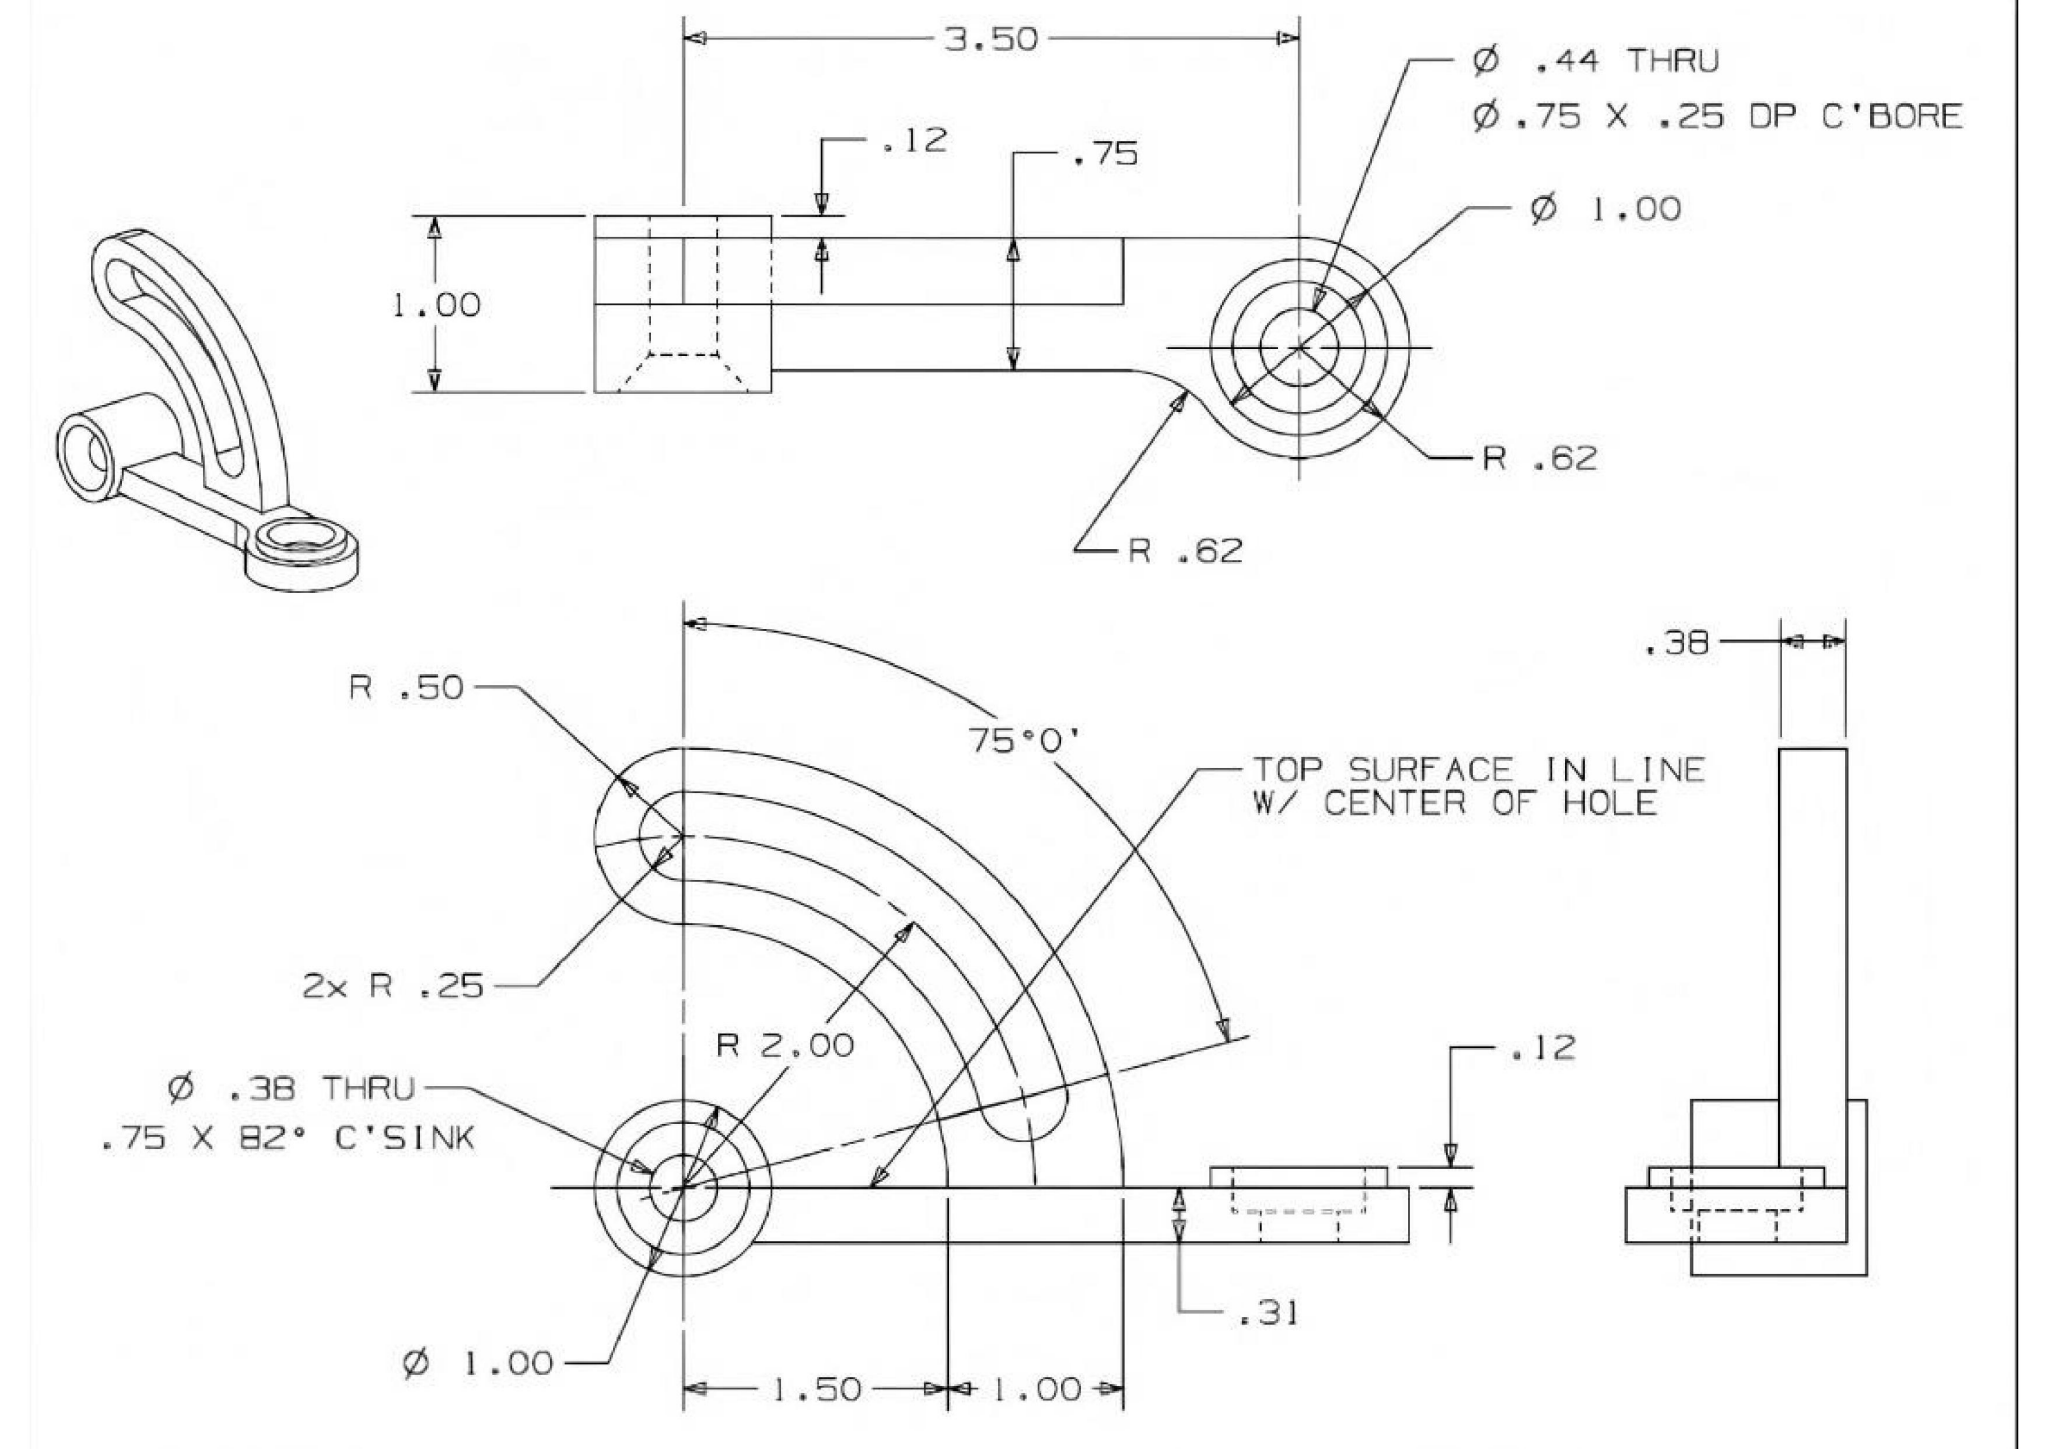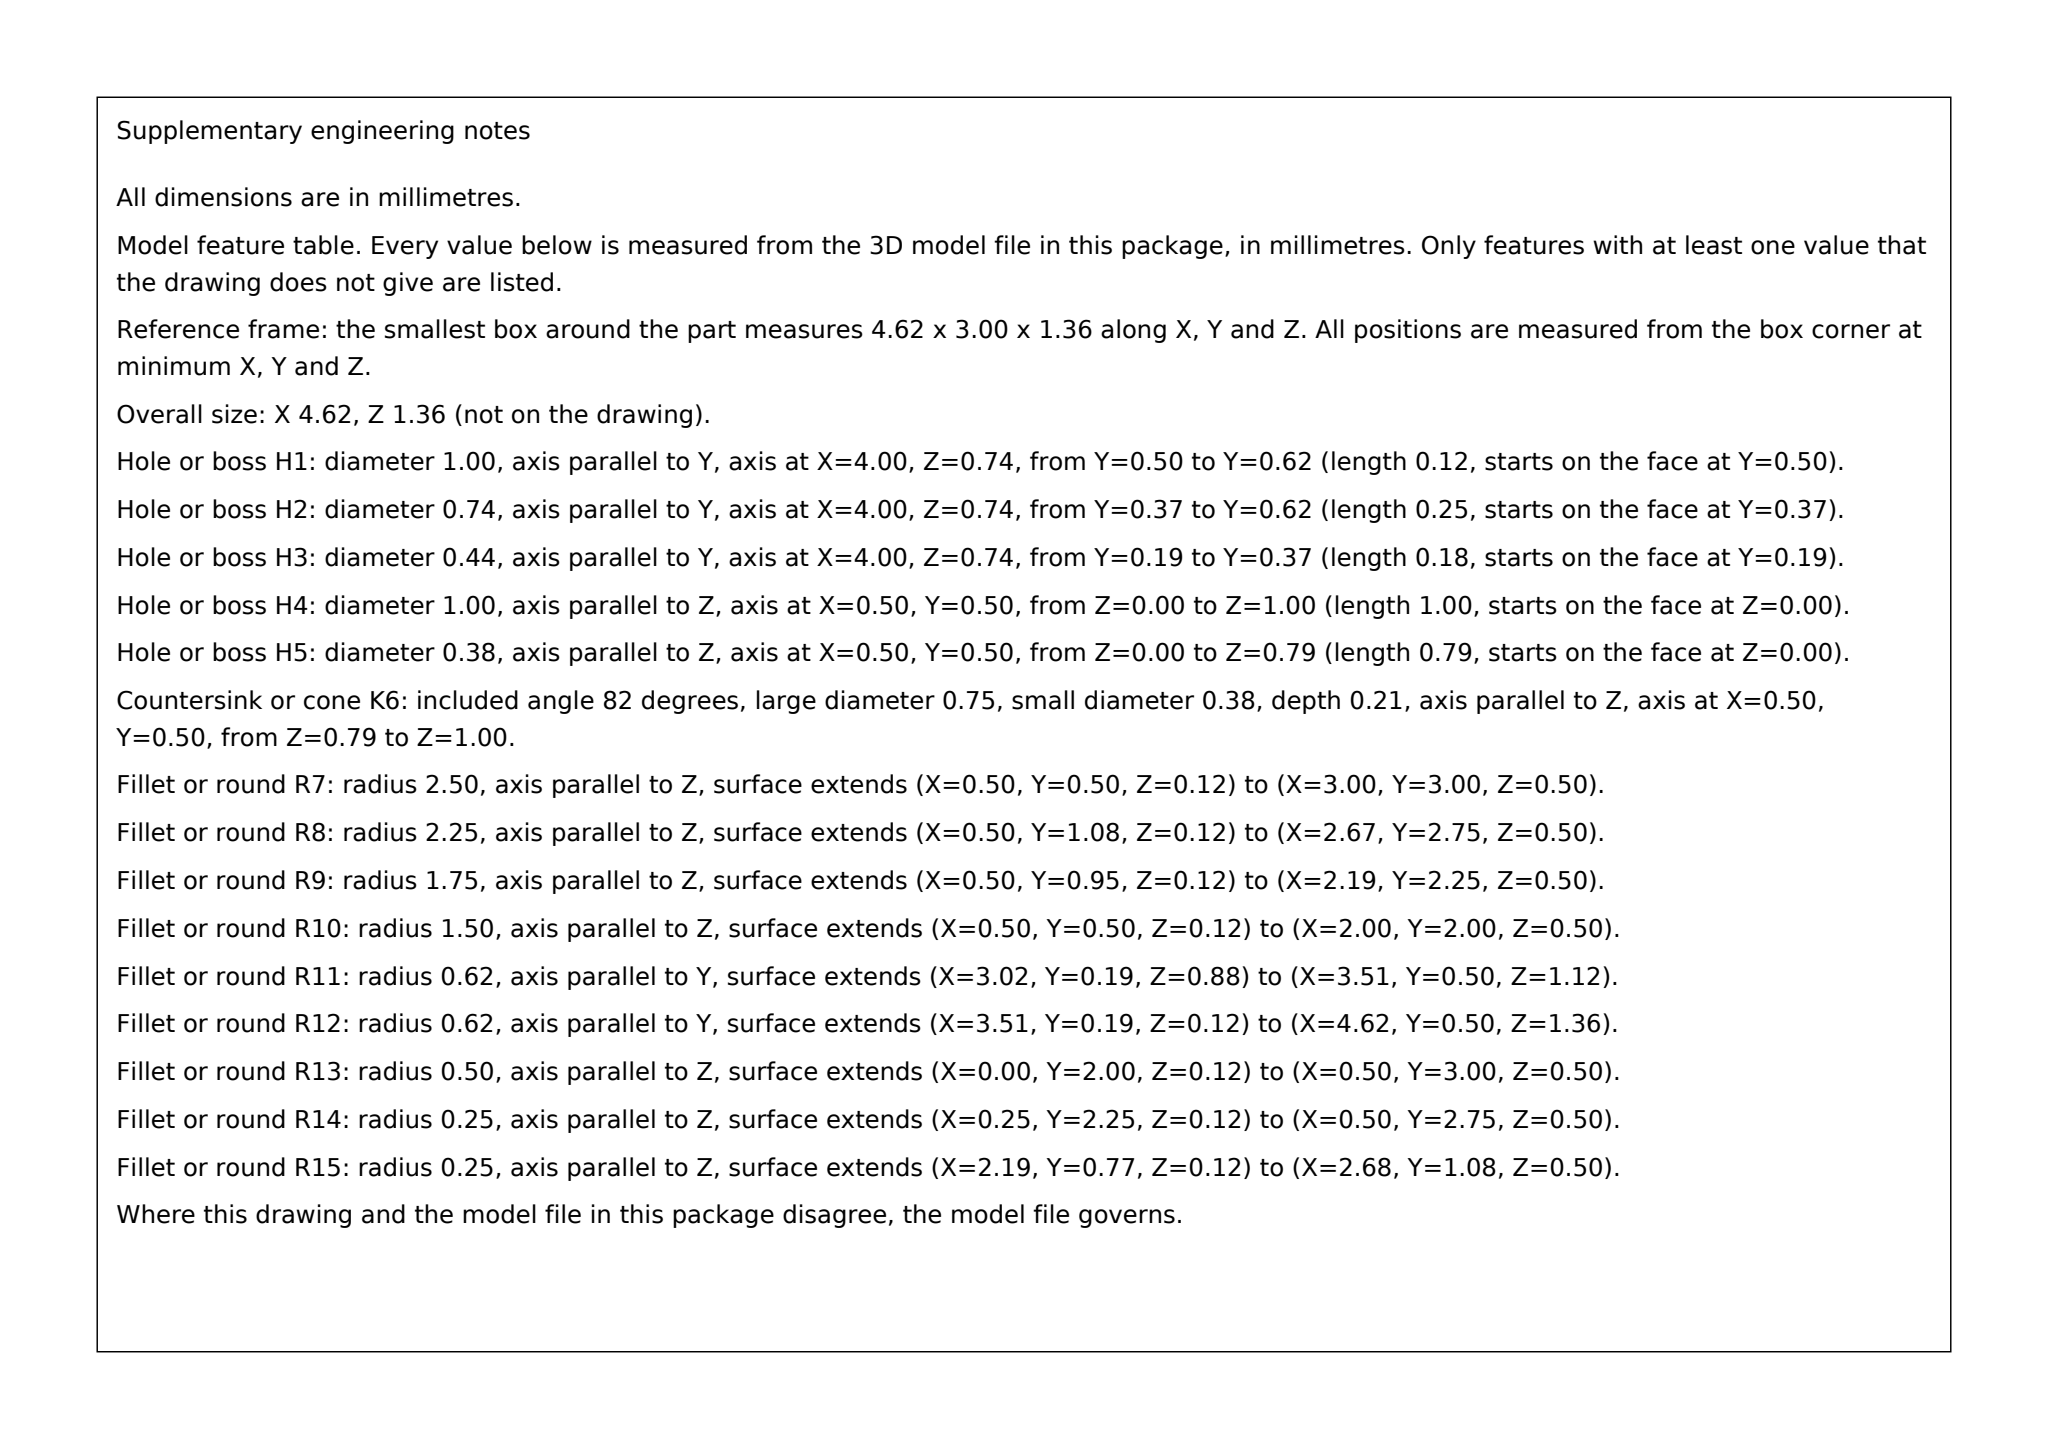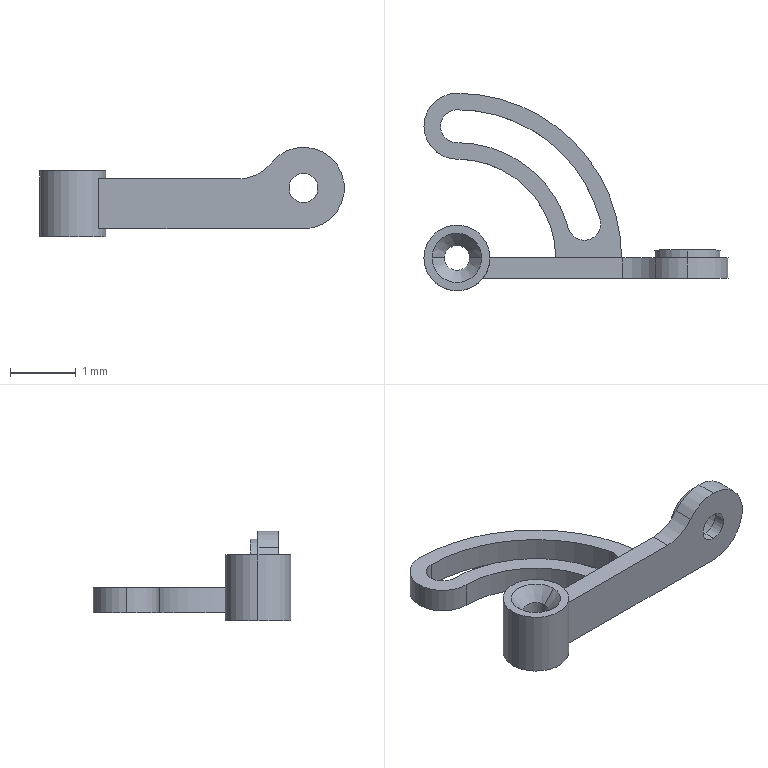Part | SolidWorks | mm | 1 solid | 33 faces | box 4.62 x 3 x 1.36 mm | volume 2 mm3 | cylinder 22 | plane 9 | cone 2 | commonest cylinder face diameters 1 x6 0.5 x3 1.24 x3 0.75 x2 0.44 x2 0.38 x2 3 x1 5 x1
build123d program:
from build123d import *

# Parameters (mm, degrees)
SKETCH1_R                                         = 0.5
BOSS_EXTRUDE1_DEPTH                               = 0.5
BOSS_EXTRUDE6_DEPTH                               = 0.31
BOSS_EXTRUDE7_START                               = -0.38
BOSS_EXTRUDE7_DEPTH                               = 0.38
SKETCH6_R                                         = 0.5
BOSS_EXTRUDE8_DEPTH                               = 0.12
F_0_38_0_38_DIAMETER_HOLE2_D                      = 0.38
F_0_38_0_38_DIAMETER_HOLE2_CSINK_D                = 0.75
F_0_38_0_38_DIAMETER_HOLE2_CSINK_ANGLE            = 82
M1_6_HEX_SOCKET_HEAD_CAP_SCREW_CBORE2_D           = 0.44
M1_6_HEX_SOCKET_HEAD_CAP_SCREW_CBORE2_CBORE_D     = 0.75
M1_6_HEX_SOCKET_HEAD_CAP_SCREW_CBORE2_CBORE_DEPTH = 0.25
CUT_EXTRUDE1_DEPTH                                = 5.895
CUT_EXTRUDE1_DEPTH_BACK                           = 5.895


with BuildPart() as part:
    # Sketch1 → Boss-Extrude1 (new, symmetric)
    with BuildSketch(Plane.XY):
        Circle(SKETCH1_R)
    extrude(amount=BOSS_EXTRUDE1_DEPTH, both=True)

    # Sketch2 → Boss-Extrude6 (add)
    with BuildSketch(Plane(origin=(0, 0, 0), x_dir=(1, 0, 0), z_dir=(0, 1, 0))):
        with BuildLine():
            Line((0, 0.38), (3.5, 0.38))
            ThreePointArc((3.5, 0.38), (4.057, -0.5128), (3.01, -0.62))
            ThreePointArc((3.01, -0.62), (2.793, -0.4432), (2.52, -0.38))
            Line((2.52, -0.38), (0, -0.38))
            Line((0, -0.38), (0, 0))
            Line((0, 0), (0, 0.38))
        make_face()
    extrude(amount=-BOSS_EXTRUDE6_DEPTH)

    # Sketch5 → Boss-Extrude7 (add)
    with BuildSketch(Plane.XY.offset(BOSS_EXTRUDE7_START)):
        with BuildLine():
            Line((2.5, 0), (1.5, 0))
            ThreePointArc((1.5, 0), (1.061, 1.061), (0, 1.5))
            ThreePointArc((0, 1.5), (-0.5, 2), (0, 2.5))
            ThreePointArc((0, 2.5), (1.768, 1.768), (2.5, 0))
        make_face()
    extrude(amount=BOSS_EXTRUDE7_DEPTH)

    # Sketch6 → Boss-Extrude8 (add)
    with BuildSketch(Plane(origin=(0, 0, 0), x_dir=(1, 0, 0), z_dir=(0, 1, 0))):
        with Locations(Location((3.5, -0.24, 0), (0, 0, 270))):
            Circle(SKETCH6_R)
    extrude(amount=BOSS_EXTRUDE8_DEPTH)

    # 0.38 _0.38_ Diameter Hole2 (through all)
    with Locations(Plane.XY.offset(0.5)):
        with Locations((0, 0)):
            CounterSinkHole(F_0_38_0_38_DIAMETER_HOLE2_D / 2, F_0_38_0_38_DIAMETER_HOLE2_CSINK_D / 2, counter_sink_angle=F_0_38_0_38_DIAMETER_HOLE2_CSINK_ANGLE)

    # M1.6 Hex Socket Head Cap Screw CBORE2 (through all)
    with Locations(Plane(origin=(0, 0.12, 0), x_dir=(1, 0, 0), z_dir=(0, 1, 0))):
        with Locations((3.5, -0.24)):
            CounterBoreHole(M1_6_HEX_SOCKET_HEAD_CAP_SCREW_CBORE2_D / 2, M1_6_HEX_SOCKET_HEAD_CAP_SCREW_CBORE2_CBORE_D / 2, M1_6_HEX_SOCKET_HEAD_CAP_SCREW_CBORE2_CBORE_DEPTH)

    # Sketch22 → Cut-Extrude1 (cut, two sides: drawn at the far end of the back side and taken through both)
    with BuildSketch(Plane.XY.offset(-CUT_EXTRUDE1_DEPTH_BACK)):
        with BuildLine():
            ThreePointArc((2.173, 0.5823), (1.37, 1.785), (0, 2.25))
            ThreePointArc((0, 2.25), (-0.25, 2), (0, 1.75))
            ThreePointArc((0, 1.75), (1.065, 1.388), (1.69, 0.4529))
            ThreePointArc((1.69, 0.4529), (1.997, 0.2762), (2.173, 0.5823))
        make_face()
    extrude(amount=CUT_EXTRUDE1_DEPTH + CUT_EXTRUDE1_DEPTH_BACK, mode=Mode.SUBTRACT)


solid = part.part